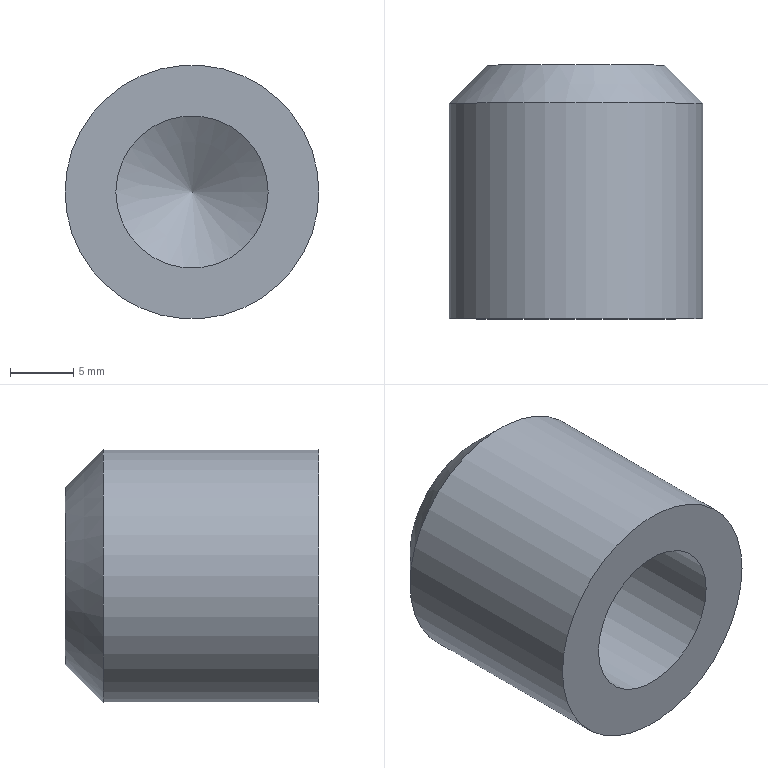Component | NX | RUBBER_PAD | 1 solid | 6 faces | box 20 x 20 x 20 mm | volume 4423 mm3 | cylinder 2 | plane 2 | cone 2 | commonest cylinder face diameters 20 x1 12 x1
STEP:
#1=CARTESIAN_POINT('',(0.,0.,0.));
#2=DIRECTION('',(0.,0.,1.));
#3=DIRECTION('',(1.,0.,0.));
#4=AXIS2_PLACEMENT_3D('',#1,#2,#3);
#5=CARTESIAN_POINT('',(10.,7.,-189.));
#6=VERTEX_POINT('',#5);
#7=CARTESIAN_POINT('',(0.,7.,-189.));
#8=DIRECTION('',(0.,-1.,0.));
#9=DIRECTION('',(1.,0.,0.));
#10=AXIS2_PLACEMENT_3D('',#7,#8,#9);
#11=CIRCLE('',#10,10.);
#12=CARTESIAN_POINT('',(0.,-10.,-189.));
#13=DIRECTION('',(0.,1.,0.));
#14=DIRECTION('',(-1.,0.,0.));
#15=AXIS2_PLACEMENT_3D('',#12,#13,#14);
#16=CYLINDRICAL_SURFACE('',#15,10.);
#17=CARTESIAN_POINT('',(9.425,17.));
#18=DIRECTION('',(-1.,0.));
#19=VECTOR('',#18,1.);
#20=LINE('',#17,#19);
#21=(GEOMETRIC_REPRESENTATION_CONTEXT(2)PARAMETRIC_REPRESENTATION_CONTEXT()REPRESENTATION_CONTEXT('',''));
#22=DEFINITIONAL_REPRESENTATION('',(#20),#21);
#23=PCURVE('',#16,#22);
#24=CARTESIAN_POINT('',(0.,7.,-189.));
#25=DIRECTION('',(0.,-1.,0.));
#26=DIRECTION('',(1.,0.,0.));
#27=AXIS2_PLACEMENT_3D('',#24,#25,#26);
#28=CONICAL_SURFACE('',#27,10.,0.7854);
#29=CARTESIAN_POINT('',(0.,0.));
#30=DIRECTION('',(1.,0.));
#31=VECTOR('',#30,1.);
#32=LINE('',#29,#31);
#33=(GEOMETRIC_REPRESENTATION_CONTEXT(2)PARAMETRIC_REPRESENTATION_CONTEXT()REPRESENTATION_CONTEXT('',''));
#34=DEFINITIONAL_REPRESENTATION('',(#32),#33);
#35=PCURVE('',#28,#34);
#36=SURFACE_CURVE('',#11,(#23,#35),.PCURVE_S1.);
#37=EDGE_CURVE('',#6,#6,#36,.T.);
#38=ORIENTED_EDGE('',*,*,#37,.T.);
#39=CARTESIAN_POINT('',(10.,-10.,-189.));
#40=VERTEX_POINT('',#39);
#41=CARTESIAN_POINT('',(10.,-10.,-189.));
#42=CARTESIAN_POINT('',(10.,7.,-189.));
#43=B_SPLINE_CURVE_WITH_KNOTS('',1,(#41,#42),.UNSPECIFIED.,.F.,.F.,(2,2),(0.,17.),.PIECEWISE_BEZIER_KNOTS.);
#44=CARTESIAN_POINT('',(3.142,0.));
#45=DIRECTION('',(0.,1.));
#46=VECTOR('',#45,1.);
#47=LINE('',#44,#46);
#48=(GEOMETRIC_REPRESENTATION_CONTEXT(2)PARAMETRIC_REPRESENTATION_CONTEXT()REPRESENTATION_CONTEXT('',''));
#49=DEFINITIONAL_REPRESENTATION('',(#47),#48);
#50=PCURVE('',#16,#49);
#51=CARTESIAN_POINT('',(9.425,0.));
#52=DIRECTION('',(0.,1.));
#53=VECTOR('',#52,1.);
#54=LINE('',#51,#53);
#55=(GEOMETRIC_REPRESENTATION_CONTEXT(2)PARAMETRIC_REPRESENTATION_CONTEXT()REPRESENTATION_CONTEXT('',''));
#56=DEFINITIONAL_REPRESENTATION('',(#54),#55);
#57=PCURVE('',#16,#56);
#58=SEAM_CURVE('',#43,(#50,#57),.PCURVE_S1.);
#59=EDGE_CURVE('',#40,#6,#58,.T.);
#60=ORIENTED_EDGE('',*,*,#59,.F.);
#61=CARTESIAN_POINT('',(0.,-10.,-189.));
#62=DIRECTION('',(0.,-1.,0.));
#63=DIRECTION('',(1.,0.,0.));
#64=AXIS2_PLACEMENT_3D('',#61,#62,#63);
#65=CIRCLE('',#64,10.);
#66=CARTESIAN_POINT('',(9.425,0.));
#67=DIRECTION('',(-1.,0.));
#68=VECTOR('',#67,1.);
#69=LINE('',#66,#68);
#70=(GEOMETRIC_REPRESENTATION_CONTEXT(2)PARAMETRIC_REPRESENTATION_CONTEXT()REPRESENTATION_CONTEXT('',''));
#71=DEFINITIONAL_REPRESENTATION('',(#69),#70);
#72=PCURVE('',#16,#71);
#73=CARTESIAN_POINT('',(0.,-10.,-189.));
#74=DIRECTION('',(0.,-1.,0.));
#75=DIRECTION('',(1.,0.,0.));
#76=AXIS2_PLACEMENT_3D('',#73,#74,#75);
#77=PLANE('',#76);
#78=CARTESIAN_POINT('',(0.,0.));
#79=DIRECTION('',(1.,0.));
#80=AXIS2_PLACEMENT_2D('',#78,#79);
#81=CIRCLE('',#80,10.);
#82=(GEOMETRIC_REPRESENTATION_CONTEXT(2)PARAMETRIC_REPRESENTATION_CONTEXT()REPRESENTATION_CONTEXT('',''));
#83=DEFINITIONAL_REPRESENTATION('',(#81),#82);
#84=PCURVE('',#77,#83);
#85=SURFACE_CURVE('',#65,(#72,#84),.PCURVE_S1.);
#86=EDGE_CURVE('',#40,#40,#85,.T.);
#87=ORIENTED_EDGE('',*,*,#86,.F.);
#88=ORIENTED_EDGE('',*,*,#59,.T.);
#89=EDGE_LOOP('',(#38,#60,#87,#88));
#90=FACE_BOUND('',#89,.T.);
#91=ADVANCED_FACE('',(#90),#16,.T.);
#92=CARTESIAN_POINT('',(-6.,-10.,-189.));
#93=VERTEX_POINT('',#92);
#94=CARTESIAN_POINT('',(0.,-10.,-189.));
#95=DIRECTION('',(0.,1.,0.));
#96=DIRECTION('',(-1.,0.,0.));
#97=AXIS2_PLACEMENT_3D('',#94,#95,#96);
#98=CIRCLE('',#97,6.);
#99=CARTESIAN_POINT('',(-6.,0.));
#100=CARTESIAN_POINT('',(-6.,10.392));
#101=CARTESIAN_POINT('',(3.,5.196));
#102=CARTESIAN_POINT('',(12.,0.));
#103=CARTESIAN_POINT('',(3.,-5.196));
#104=CARTESIAN_POINT('',(-6.,-10.392));
#105=CARTESIAN_POINT('',(-6.,0.));
#106=(BOUNDED_CURVE()B_SPLINE_CURVE(2,(#99,#100,#101,#102,#103,#104,#105),.UNSPECIFIED.,.T.,.F.)B_SPLINE_CURVE_WITH_KNOTS((1,2,2,2,2,1),(-2.094,0.,2.094,4.189,6.283,8.378),.UNSPECIFIED.)CURVE()GEOMETRIC_REPRESENTATION_ITEM()RATIONAL_B_SPLINE_CURVE((1.,0.5,1.,0.5,1.,0.5,1.))REPRESENTATION_ITEM(''));
#107=(GEOMETRIC_REPRESENTATION_CONTEXT(2)PARAMETRIC_REPRESENTATION_CONTEXT()REPRESENTATION_CONTEXT('',''));
#108=DEFINITIONAL_REPRESENTATION('',(#106),#107);
#109=PCURVE('',#77,#108);
#110=CARTESIAN_POINT('',(0.,-10.,-189.));
#111=DIRECTION('',(0.,1.,0.));
#112=DIRECTION('',(-1.,0.,0.));
#113=AXIS2_PLACEMENT_3D('',#110,#111,#112);
#114=CYLINDRICAL_SURFACE('',#113,6.);
#115=CARTESIAN_POINT('',(0.,0.));
#116=DIRECTION('',(1.,0.));
#117=VECTOR('',#116,1.);
#118=LINE('',#115,#117);
#119=(GEOMETRIC_REPRESENTATION_CONTEXT(2)PARAMETRIC_REPRESENTATION_CONTEXT()REPRESENTATION_CONTEXT('',''));
#120=DEFINITIONAL_REPRESENTATION('',(#118),#119);
#121=PCURVE('',#114,#120);
#122=SURFACE_CURVE('',#98,(#109,#121),.PCURVE_S1.);
#123=EDGE_CURVE('',#93,#93,#122,.T.);
#124=ORIENTED_EDGE('',*,*,#123,.T.);
#125=EDGE_LOOP('',(#124));
#126=FACE_BOUND('',#125,.T.);
#127=ORIENTED_EDGE('',*,*,#86,.T.);
#128=EDGE_LOOP('',(#127));
#129=FACE_BOUND('',#128,.T.);
#130=ADVANCED_FACE('',(#126,#129),#77,.T.);
#131=CARTESIAN_POINT('',(7.,10.,-189.));
#132=VERTEX_POINT('',#131);
#133=CARTESIAN_POINT('',(0.,10.,-189.));
#134=DIRECTION('',(0.,1.,0.));
#135=DIRECTION('',(1.,0.,0.));
#136=AXIS2_PLACEMENT_3D('',#133,#134,#135);
#137=CIRCLE('',#136,7.);
#138=CARTESIAN_POINT('',(0.,10.,-189.));
#139=DIRECTION('',(0.,-1.,0.));
#140=DIRECTION('',(1.,0.,0.));
#141=AXIS2_PLACEMENT_3D('',#138,#139,#140);
#142=PLANE('',#141);
#143=CARTESIAN_POINT('',(7.,0.));
#144=CARTESIAN_POINT('',(7.,-12.124));
#145=CARTESIAN_POINT('',(-3.5,-6.062));
#146=CARTESIAN_POINT('',(-14.,-0.));
#147=CARTESIAN_POINT('',(-3.5,6.062));
#148=CARTESIAN_POINT('',(7.,12.124));
#149=CARTESIAN_POINT('',(7.,0.));
#150=(BOUNDED_CURVE()B_SPLINE_CURVE(2,(#143,#144,#145,#146,#147,#148,#149),.UNSPECIFIED.,.T.,.F.)B_SPLINE_CURVE_WITH_KNOTS((1,2,2,2,2,1),(-2.094,0.,2.094,4.189,6.283,8.378),.UNSPECIFIED.)CURVE()GEOMETRIC_REPRESENTATION_ITEM()RATIONAL_B_SPLINE_CURVE((1.,0.5,1.,0.5,1.,0.5,1.))REPRESENTATION_ITEM(''));
#151=(GEOMETRIC_REPRESENTATION_CONTEXT(2)PARAMETRIC_REPRESENTATION_CONTEXT()REPRESENTATION_CONTEXT('',''));
#152=DEFINITIONAL_REPRESENTATION('',(#150),#151);
#153=PCURVE('',#142,#152);
#154=CARTESIAN_POINT('',(6.283,-3.));
#155=DIRECTION('',(-1.,0.));
#156=VECTOR('',#155,1.);
#157=LINE('',#154,#156);
#158=(GEOMETRIC_REPRESENTATION_CONTEXT(2)PARAMETRIC_REPRESENTATION_CONTEXT()REPRESENTATION_CONTEXT('',''));
#159=DEFINITIONAL_REPRESENTATION('',(#157),#158);
#160=PCURVE('',#28,#159);
#161=SURFACE_CURVE('',#137,(#153,#160),.PCURVE_S1.);
#162=EDGE_CURVE('',#132,#132,#161,.T.);
#163=ORIENTED_EDGE('',*,*,#162,.T.);
#164=EDGE_LOOP('',(#163));
#165=FACE_BOUND('',#164,.T.);
#166=ADVANCED_FACE('',(#165),#142,.F.);
#167=ORIENTED_EDGE('',*,*,#162,.F.);
#168=CARTESIAN_POINT('',(7.,10.,-189.));
#169=CARTESIAN_POINT('',(10.,7.,-189.));
#170=B_SPLINE_CURVE_WITH_KNOTS('',1,(#168,#169),.UNSPECIFIED.,.F.,.F.,(2,2),(-4.243,0.),.PIECEWISE_BEZIER_KNOTS.);
#171=CARTESIAN_POINT('',(6.283,0.));
#172=DIRECTION('',(0.,1.));
#173=VECTOR('',#172,1.);
#174=LINE('',#171,#173);
#175=(GEOMETRIC_REPRESENTATION_CONTEXT(2)PARAMETRIC_REPRESENTATION_CONTEXT()REPRESENTATION_CONTEXT('',''));
#176=DEFINITIONAL_REPRESENTATION('',(#174),#175);
#177=PCURVE('',#28,#176);
#178=CARTESIAN_POINT('',(0.,0.));
#179=DIRECTION('',(0.,1.));
#180=VECTOR('',#179,1.);
#181=LINE('',#178,#180);
#182=(GEOMETRIC_REPRESENTATION_CONTEXT(2)PARAMETRIC_REPRESENTATION_CONTEXT()REPRESENTATION_CONTEXT('',''));
#183=DEFINITIONAL_REPRESENTATION('',(#181),#182);
#184=PCURVE('',#28,#183);
#185=SEAM_CURVE('',#170,(#177,#184),.PCURVE_S1.);
#186=EDGE_CURVE('',#132,#6,#185,.T.);
#187=ORIENTED_EDGE('',*,*,#186,.T.);
#188=ORIENTED_EDGE('',*,*,#37,.F.);
#189=ORIENTED_EDGE('',*,*,#186,.F.);
#190=EDGE_LOOP('',(#167,#187,#188,#189));
#191=FACE_BOUND('',#190,.T.);
#192=ADVANCED_FACE('',(#191),#28,.T.);
#193=CARTESIAN_POINT('',(6.,3.,-189.));
#194=VERTEX_POINT('',#193);
#195=CARTESIAN_POINT('',(-6.,3.,-189.));
#196=VERTEX_POINT('',#195);
#197=CARTESIAN_POINT('',(0.,3.,-189.));
#198=DIRECTION('',(0.,-1.,0.));
#199=DIRECTION('',(-1.,0.,0.));
#200=AXIS2_PLACEMENT_3D('',#197,#198,#199);
#201=CIRCLE('',#200,6.);
#202=CARTESIAN_POINT('',(0.,3.,-189.));
#203=DIRECTION('',(0.,-1.,0.));
#204=DIRECTION('',(1.,0.,0.));
#205=AXIS2_PLACEMENT_3D('',#202,#203,#204);
#206=CONICAL_SURFACE('',#205,6.,1.03);
#207=CARTESIAN_POINT('',(-3.142,0.));
#208=DIRECTION('',(1.,0.));
#209=VECTOR('',#208,1.);
#210=LINE('',#207,#209);
#211=(GEOMETRIC_REPRESENTATION_CONTEXT(2)PARAMETRIC_REPRESENTATION_CONTEXT()REPRESENTATION_CONTEXT('',''));
#212=DEFINITIONAL_REPRESENTATION('',(#210),#211);
#213=PCURVE('',#206,#212);
#214=CARTESIAN_POINT('',(6.283,13.));
#215=DIRECTION('',(-1.,0.));
#216=VECTOR('',#215,1.);
#217=LINE('',#214,#216);
#218=(GEOMETRIC_REPRESENTATION_CONTEXT(2)PARAMETRIC_REPRESENTATION_CONTEXT()REPRESENTATION_CONTEXT('',''));
#219=DEFINITIONAL_REPRESENTATION('',(#217),#218);
#220=PCURVE('',#114,#219);
#221=SURFACE_CURVE('',#201,(#213,#220),.PCURVE_S1.);
#222=EDGE_CURVE('',#194,#196,#221,.T.);
#223=ORIENTED_EDGE('',*,*,#222,.F.);
#224=CARTESIAN_POINT('',(0.,6.605,-189.));
#225=VERTEX_POINT('',#224);
#226=CARTESIAN_POINT('',(0.,6.605,-189.));
#227=CARTESIAN_POINT('',(6.,3.,-189.));
#228=B_SPLINE_CURVE_WITH_KNOTS('',1,(#226,#227),.UNSPECIFIED.,.F.,.F.,(2,2),(-7.,0.),.PIECEWISE_BEZIER_KNOTS.);
#229=CARTESIAN_POINT('',(0.,0.));
#230=DIRECTION('',(0.,1.));
#231=VECTOR('',#230,1.);
#232=LINE('',#229,#231);
#233=(GEOMETRIC_REPRESENTATION_CONTEXT(2)PARAMETRIC_REPRESENTATION_CONTEXT()REPRESENTATION_CONTEXT('',''));
#234=DEFINITIONAL_REPRESENTATION('',(#232),#233);
#235=PCURVE('',#206,#234);
#236=CARTESIAN_POINT('',(6.283,0.));
#237=DIRECTION('',(0.,1.));
#238=VECTOR('',#237,1.);
#239=LINE('',#236,#238);
#240=(GEOMETRIC_REPRESENTATION_CONTEXT(2)PARAMETRIC_REPRESENTATION_CONTEXT()REPRESENTATION_CONTEXT('',''));
#241=DEFINITIONAL_REPRESENTATION('',(#239),#240);
#242=PCURVE('',#206,#241);
#243=SEAM_CURVE('',#228,(#235,#242),.PCURVE_S1.);
#244=EDGE_CURVE('',#225,#194,#243,.T.);
#245=ORIENTED_EDGE('',*,*,#244,.F.);
#246=ORIENTED_EDGE('',*,*,#244,.T.);
#247=CARTESIAN_POINT('',(0.,3.,-189.));
#248=DIRECTION('',(0.,-1.,0.));
#249=DIRECTION('',(-1.,0.,0.));
#250=AXIS2_PLACEMENT_3D('',#247,#248,#249);
#251=CIRCLE('',#250,6.);
#252=CARTESIAN_POINT('',(3.142,0.));
#253=DIRECTION('',(1.,0.));
#254=VECTOR('',#253,1.);
#255=LINE('',#252,#254);
#256=(GEOMETRIC_REPRESENTATION_CONTEXT(2)PARAMETRIC_REPRESENTATION_CONTEXT()REPRESENTATION_CONTEXT('',''));
#257=DEFINITIONAL_REPRESENTATION('',(#255),#256);
#258=PCURVE('',#206,#257);
#259=CARTESIAN_POINT('',(6.283,13.));
#260=DIRECTION('',(-1.,0.));
#261=VECTOR('',#260,1.);
#262=LINE('',#259,#261);
#263=(GEOMETRIC_REPRESENTATION_CONTEXT(2)PARAMETRIC_REPRESENTATION_CONTEXT()REPRESENTATION_CONTEXT('',''));
#264=DEFINITIONAL_REPRESENTATION('',(#262),#263);
#265=PCURVE('',#114,#264);
#266=SURFACE_CURVE('',#251,(#258,#265),.PCURVE_S1.);
#267=EDGE_CURVE('',#196,#194,#266,.T.);
#268=ORIENTED_EDGE('',*,*,#267,.F.);
#269=EDGE_LOOP('',(#223,#245,#246,#268));
#270=FACE_BOUND('',#269,.F.);
#271=ADVANCED_FACE('',(#270),#206,.F.);
#272=ORIENTED_EDGE('',*,*,#222,.T.);
#273=CARTESIAN_POINT('',(-6.,-10.,-189.));
#274=CARTESIAN_POINT('',(-6.,3.,-189.));
#275=B_SPLINE_CURVE_WITH_KNOTS('',1,(#273,#274),.UNSPECIFIED.,.F.,.F.,(2,2),(0.,13.),.PIECEWISE_BEZIER_KNOTS.);
#276=CARTESIAN_POINT('',(0.,0.));
#277=DIRECTION('',(0.,1.));
#278=VECTOR('',#277,1.);
#279=LINE('',#276,#278);
#280=(GEOMETRIC_REPRESENTATION_CONTEXT(2)PARAMETRIC_REPRESENTATION_CONTEXT()REPRESENTATION_CONTEXT('',''));
#281=DEFINITIONAL_REPRESENTATION('',(#279),#280);
#282=PCURVE('',#114,#281);
#283=CARTESIAN_POINT('',(6.283,0.));
#284=DIRECTION('',(0.,1.));
#285=VECTOR('',#284,1.);
#286=LINE('',#283,#285);
#287=(GEOMETRIC_REPRESENTATION_CONTEXT(2)PARAMETRIC_REPRESENTATION_CONTEXT()REPRESENTATION_CONTEXT('',''));
#288=DEFINITIONAL_REPRESENTATION('',(#286),#287);
#289=PCURVE('',#114,#288);
#290=SEAM_CURVE('',#275,(#282,#289),.PCURVE_S1.);
#291=EDGE_CURVE('',#93,#196,#290,.T.);
#292=ORIENTED_EDGE('',*,*,#291,.F.);
#293=ORIENTED_EDGE('',*,*,#123,.T.);
#294=ORIENTED_EDGE('',*,*,#291,.T.);
#295=ORIENTED_EDGE('',*,*,#267,.T.);
#296=EDGE_LOOP('',(#272,#292,#293,#294,#295));
#297=FACE_BOUND('',#296,.F.);
#298=ADVANCED_FACE('',(#297),#114,.F.);
#299=CLOSED_SHELL('',(#91,#130,#166,#192,#271,#298));
#300=MANIFOLD_SOLID_BREP('',#299);
#301=(LENGTH_UNIT()NAMED_UNIT(*)SI_UNIT(.MILLI.,.METRE.));
#302=UNCERTAINTY_MEASURE_WITH_UNIT(LENGTH_MEASURE(0.00001),#301,'','');
#303=(NAMED_UNIT(*)PLANE_ANGLE_UNIT()SI_UNIT($,.RADIAN.));
#304=(NAMED_UNIT(*)SI_UNIT($,.STERADIAN.)SOLID_ANGLE_UNIT());
#305=(GEOMETRIC_REPRESENTATION_CONTEXT(3)GLOBAL_UNCERTAINTY_ASSIGNED_CONTEXT((#302))GLOBAL_UNIT_ASSIGNED_CONTEXT((#301,#303,#304))REPRESENTATION_CONTEXT('',''));
#306=ADVANCED_BREP_SHAPE_REPRESENTATION('',(#4,#300),#305);